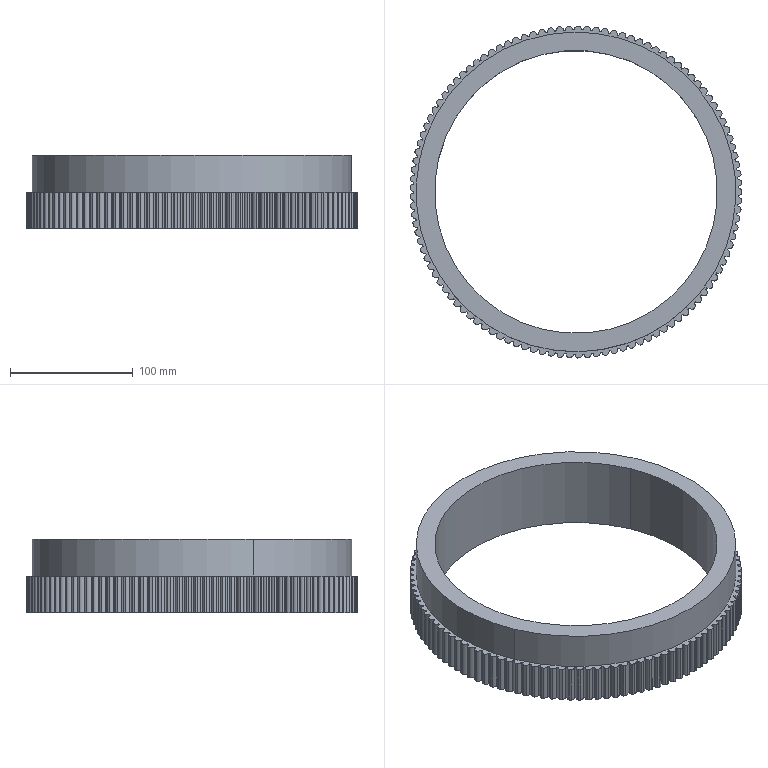Component | SolidWorks | SlewingBearing-1 | 1 solid | 497 faces | volume 789551 mm3 | cylinder 494 | plane 3 | commonest cylinder face diameters 7.458 x263 270 x114 264 x113 230 x2 260 x2 | material 45